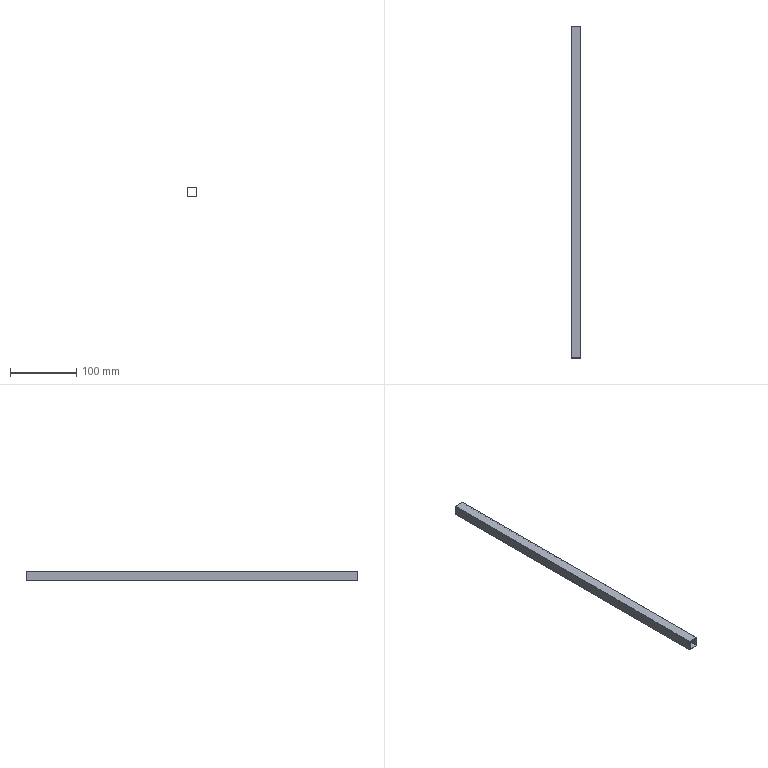Component | SolidWorks | Column-2 | 1 solid | 10 faces | box 15 x 500 x 15 mm | volume 28000 mm3 | plane 10
build123d program:
from build123d import *

# Parameters (mm, degrees)
SKETCH1_W           = 15
SKETCH1_H           = 15
SKETCH1_W_2         = 13
SKETCH1_H_2         = 13
BOSS_EXTRUDE1_DEPTH = 500


with BuildPart() as part:
    # Sketch1 → Boss-Extrude1 (new body)
    with BuildSketch(Plane(origin=(0, 0, 0), x_dir=(1, 0, 0), z_dir=(0, 1, 0))):
        Rectangle(SKETCH1_W, SKETCH1_H)
        Rectangle(SKETCH1_W_2, SKETCH1_H_2, mode=Mode.SUBTRACT)
    extrude(amount=BOSS_EXTRUDE1_DEPTH)


solid = part.part

# Placed as in the assembly
solid = solid.moved(Location((75.741, -541.715, 1459.224), (0, 0, 0)))
STEP:
#1=COLOUR_RGB('',0.7922,0.8196,0.9333);
#2=FILL_AREA_STYLE_COLOUR('',#1);
#3=FILL_AREA_STYLE('',(#2));
#4=SURFACE_STYLE_FILL_AREA(#3);
#5=SURFACE_SIDE_STYLE('',(#4));
#6=SURFACE_STYLE_USAGE(.BOTH.,#5);
#7=PRESENTATION_STYLE_ASSIGNMENT((#6));
#8=CARTESIAN_POINT('',(2.687,-1.642,57.155));
#9=VERTEX_POINT('',#8);
#10=CARTESIAN_POINT('',(2.687,-1.642,57.745));
#11=VERTEX_POINT('',#10);
#12=CARTESIAN_POINT('',(2.687,-1.642,57.155));
#13=DIRECTION('',(0.,0.,1.));
#14=VECTOR('',#13,39.37);
#15=LINE('',#12,#14);
#16=EDGE_CURVE('',#9,#11,#15,.T.);
#17=ORIENTED_EDGE('',*,*,#16,.T.);
#18=CARTESIAN_POINT('',(3.277,-1.642,57.745));
#19=VERTEX_POINT('',#18);
#20=CARTESIAN_POINT('',(3.277,-1.642,57.745));
#21=DIRECTION('',(1.,0.,0.));
#22=VECTOR('',#21,39.37);
#23=LINE('',#20,#22);
#24=EDGE_CURVE('',#11,#19,#23,.T.);
#25=ORIENTED_EDGE('',*,*,#24,.T.);
#26=CARTESIAN_POINT('',(3.277,-1.642,57.155));
#27=VERTEX_POINT('',#26);
#28=CARTESIAN_POINT('',(3.277,-1.642,57.155));
#29=DIRECTION('',(0.,0.,-1.));
#30=VECTOR('',#29,39.37);
#31=LINE('',#28,#30);
#32=EDGE_CURVE('',#19,#27,#31,.T.);
#33=ORIENTED_EDGE('',*,*,#32,.T.);
#34=CARTESIAN_POINT('',(3.277,-1.642,57.155));
#35=DIRECTION('',(-1.,0.,0.));
#36=VECTOR('',#35,39.37);
#37=LINE('',#34,#36);
#38=EDGE_CURVE('',#27,#9,#37,.T.);
#39=ORIENTED_EDGE('',*,*,#38,.T.);
#40=EDGE_LOOP('',(#17,#25,#33,#39));
#41=FACE_OUTER_BOUND('',#40,.T.);
#42=CARTESIAN_POINT('',(3.238,-1.642,57.706));
#43=VERTEX_POINT('',#42);
#44=CARTESIAN_POINT('',(3.238,-1.642,57.194));
#45=VERTEX_POINT('',#44);
#46=CARTESIAN_POINT('',(3.238,-1.642,57.194));
#47=DIRECTION('',(0.,0.,-1.));
#48=VECTOR('',#47,39.37);
#49=LINE('',#46,#48);
#50=EDGE_CURVE('',#43,#45,#49,.T.);
#51=ORIENTED_EDGE('',*,*,#50,.F.);
#52=CARTESIAN_POINT('',(2.726,-1.642,57.706));
#53=VERTEX_POINT('',#52);
#54=CARTESIAN_POINT('',(2.726,-1.642,57.706));
#55=DIRECTION('',(1.,0.,0.));
#56=VECTOR('',#55,39.37);
#57=LINE('',#54,#56);
#58=EDGE_CURVE('',#53,#43,#57,.T.);
#59=ORIENTED_EDGE('',*,*,#58,.F.);
#60=CARTESIAN_POINT('',(2.726,-1.642,57.194));
#61=VERTEX_POINT('',#60);
#62=CARTESIAN_POINT('',(2.726,-1.642,57.194));
#63=DIRECTION('',(0.,0.,1.));
#64=VECTOR('',#63,39.37);
#65=LINE('',#62,#64);
#66=EDGE_CURVE('',#61,#53,#65,.T.);
#67=ORIENTED_EDGE('',*,*,#66,.F.);
#68=CARTESIAN_POINT('',(2.726,-1.642,57.194));
#69=DIRECTION('',(-1.,0.,-0.));
#70=VECTOR('',#69,39.37);
#71=LINE('',#68,#70);
#72=EDGE_CURVE('',#45,#61,#71,.T.);
#73=ORIENTED_EDGE('',*,*,#72,.F.);
#74=EDGE_LOOP('',(#51,#59,#67,#73));
#75=FACE_BOUND('',#74,.T.);
#76=CARTESIAN_POINT('',(2.982,-1.642,57.45));
#77=DIRECTION('',(0.,-1.,0.));
#78=DIRECTION('',(0.,0.,1.));
#79=AXIS2_PLACEMENT_3D('',#76,#77,#78);
#80=PLANE('',#79);
#81=ADVANCED_FACE('',(#41,#75),#80,.F.);
#82=CARTESIAN_POINT('',(2.687,-21.327,57.155));
#83=VERTEX_POINT('',#82);
#84=CARTESIAN_POINT('',(2.687,-21.327,57.745));
#85=VERTEX_POINT('',#84);
#86=CARTESIAN_POINT('',(2.687,-21.327,57.155));
#87=DIRECTION('',(0.,0.,1.));
#88=VECTOR('',#87,39.37);
#89=LINE('',#86,#88);
#90=EDGE_CURVE('',#83,#85,#89,.T.);
#91=ORIENTED_EDGE('',*,*,#90,.F.);
#92=CARTESIAN_POINT('',(3.277,-21.327,57.155));
#93=VERTEX_POINT('',#92);
#94=CARTESIAN_POINT('',(3.277,-21.327,57.155));
#95=DIRECTION('',(-1.,0.,0.));
#96=VECTOR('',#95,39.37);
#97=LINE('',#94,#96);
#98=EDGE_CURVE('',#93,#83,#97,.T.);
#99=ORIENTED_EDGE('',*,*,#98,.F.);
#100=CARTESIAN_POINT('',(3.277,-21.327,57.745));
#101=VERTEX_POINT('',#100);
#102=CARTESIAN_POINT('',(3.277,-21.327,57.155));
#103=DIRECTION('',(0.,0.,-1.));
#104=VECTOR('',#103,39.37);
#105=LINE('',#102,#104);
#106=EDGE_CURVE('',#101,#93,#105,.T.);
#107=ORIENTED_EDGE('',*,*,#106,.F.);
#108=CARTESIAN_POINT('',(3.277,-21.327,57.745));
#109=DIRECTION('',(1.,0.,0.));
#110=VECTOR('',#109,39.37);
#111=LINE('',#108,#110);
#112=EDGE_CURVE('',#85,#101,#111,.T.);
#113=ORIENTED_EDGE('',*,*,#112,.F.);
#114=EDGE_LOOP('',(#91,#99,#107,#113));
#115=FACE_OUTER_BOUND('',#114,.T.);
#116=CARTESIAN_POINT('',(2.726,-21.327,57.706));
#117=VERTEX_POINT('',#116);
#118=CARTESIAN_POINT('',(3.238,-21.327,57.706));
#119=VERTEX_POINT('',#118);
#120=CARTESIAN_POINT('',(2.726,-21.327,57.706));
#121=DIRECTION('',(1.,0.,0.));
#122=VECTOR('',#121,39.37);
#123=LINE('',#120,#122);
#124=EDGE_CURVE('',#117,#119,#123,.T.);
#125=ORIENTED_EDGE('',*,*,#124,.T.);
#126=CARTESIAN_POINT('',(3.238,-21.327,57.194));
#127=VERTEX_POINT('',#126);
#128=CARTESIAN_POINT('',(3.238,-21.327,57.194));
#129=DIRECTION('',(0.,0.,-1.));
#130=VECTOR('',#129,39.37);
#131=LINE('',#128,#130);
#132=EDGE_CURVE('',#119,#127,#131,.T.);
#133=ORIENTED_EDGE('',*,*,#132,.T.);
#134=CARTESIAN_POINT('',(2.726,-21.327,57.194));
#135=VERTEX_POINT('',#134);
#136=CARTESIAN_POINT('',(2.726,-21.327,57.194));
#137=DIRECTION('',(-1.,0.,-0.));
#138=VECTOR('',#137,39.37);
#139=LINE('',#136,#138);
#140=EDGE_CURVE('',#127,#135,#139,.T.);
#141=ORIENTED_EDGE('',*,*,#140,.T.);
#142=CARTESIAN_POINT('',(2.726,-21.327,57.194));
#143=DIRECTION('',(0.,0.,1.));
#144=VECTOR('',#143,39.37);
#145=LINE('',#142,#144);
#146=EDGE_CURVE('',#135,#117,#145,.T.);
#147=ORIENTED_EDGE('',*,*,#146,.T.);
#148=EDGE_LOOP('',(#125,#133,#141,#147));
#149=FACE_BOUND('',#148,.T.);
#150=CARTESIAN_POINT('',(2.982,-21.327,57.45));
#151=DIRECTION('',(0.,-1.,0.));
#152=DIRECTION('',(0.,0.,1.));
#153=AXIS2_PLACEMENT_3D('',#150,#151,#152);
#154=PLANE('',#153);
#155=ADVANCED_FACE('',(#115,#149),#154,.T.);
#156=ORIENTED_EDGE('',*,*,#90,.T.);
#157=CARTESIAN_POINT('',(2.687,-1.642,57.745));
#158=DIRECTION('',(0.,-1.,0.));
#159=VECTOR('',#158,39.37);
#160=LINE('',#157,#159);
#161=EDGE_CURVE('',#11,#85,#160,.T.);
#162=ORIENTED_EDGE('',*,*,#161,.F.);
#163=ORIENTED_EDGE('',*,*,#16,.F.);
#164=CARTESIAN_POINT('',(2.687,-1.642,57.155));
#165=DIRECTION('',(0.,-1.,0.));
#166=VECTOR('',#165,39.37);
#167=LINE('',#164,#166);
#168=EDGE_CURVE('',#9,#83,#167,.T.);
#169=ORIENTED_EDGE('',*,*,#168,.T.);
#170=EDGE_LOOP('',(#156,#162,#163,#169));
#171=FACE_OUTER_BOUND('',#170,.T.);
#172=CARTESIAN_POINT('',(2.687,-1.642,57.155));
#173=DIRECTION('',(1.,0.,0.));
#174=DIRECTION('',(0.,0.,-1.));
#175=AXIS2_PLACEMENT_3D('',#172,#173,#174);
#176=PLANE('',#175);
#177=ADVANCED_FACE('',(#171),#176,.F.);
#178=ORIENTED_EDGE('',*,*,#112,.T.);
#179=CARTESIAN_POINT('',(3.277,-1.642,57.745));
#180=DIRECTION('',(0.,-1.,0.));
#181=VECTOR('',#180,39.37);
#182=LINE('',#179,#181);
#183=EDGE_CURVE('',#19,#101,#182,.T.);
#184=ORIENTED_EDGE('',*,*,#183,.F.);
#185=ORIENTED_EDGE('',*,*,#24,.F.);
#186=ORIENTED_EDGE('',*,*,#161,.T.);
#187=EDGE_LOOP('',(#178,#184,#185,#186));
#188=FACE_OUTER_BOUND('',#187,.T.);
#189=CARTESIAN_POINT('',(3.277,-1.642,57.745));
#190=DIRECTION('',(0.,0.,-1.));
#191=DIRECTION('',(-1.,0.,0.));
#192=AXIS2_PLACEMENT_3D('',#189,#190,#191);
#193=PLANE('',#192);
#194=ADVANCED_FACE('',(#188),#193,.F.);
#195=ORIENTED_EDGE('',*,*,#106,.T.);
#196=CARTESIAN_POINT('',(3.277,-1.642,57.155));
#197=DIRECTION('',(0.,-1.,0.));
#198=VECTOR('',#197,39.37);
#199=LINE('',#196,#198);
#200=EDGE_CURVE('',#27,#93,#199,.T.);
#201=ORIENTED_EDGE('',*,*,#200,.F.);
#202=ORIENTED_EDGE('',*,*,#32,.F.);
#203=ORIENTED_EDGE('',*,*,#183,.T.);
#204=EDGE_LOOP('',(#195,#201,#202,#203));
#205=FACE_OUTER_BOUND('',#204,.T.);
#206=CARTESIAN_POINT('',(3.277,-1.642,57.155));
#207=DIRECTION('',(-1.,0.,0.));
#208=DIRECTION('',(0.,0.,1.));
#209=AXIS2_PLACEMENT_3D('',#206,#207,#208);
#210=PLANE('',#209);
#211=ADVANCED_FACE('',(#205),#210,.F.);
#212=ORIENTED_EDGE('',*,*,#98,.T.);
#213=ORIENTED_EDGE('',*,*,#168,.F.);
#214=ORIENTED_EDGE('',*,*,#38,.F.);
#215=ORIENTED_EDGE('',*,*,#200,.T.);
#216=EDGE_LOOP('',(#212,#213,#214,#215));
#217=FACE_OUTER_BOUND('',#216,.T.);
#218=CARTESIAN_POINT('',(3.277,-1.642,57.155));
#219=DIRECTION('',(0.,0.,1.));
#220=DIRECTION('',(1.,0.,0.));
#221=AXIS2_PLACEMENT_3D('',#218,#219,#220);
#222=PLANE('',#221);
#223=ADVANCED_FACE('',(#217),#222,.F.);
#224=ORIENTED_EDGE('',*,*,#132,.F.);
#225=CARTESIAN_POINT('',(3.238,-1.642,57.706));
#226=DIRECTION('',(0.,-1.,0.));
#227=VECTOR('',#226,39.37);
#228=LINE('',#225,#227);
#229=EDGE_CURVE('',#43,#119,#228,.T.);
#230=ORIENTED_EDGE('',*,*,#229,.F.);
#231=ORIENTED_EDGE('',*,*,#50,.T.);
#232=CARTESIAN_POINT('',(3.238,-1.642,57.194));
#233=DIRECTION('',(0.,-1.,0.));
#234=VECTOR('',#233,39.37);
#235=LINE('',#232,#234);
#236=EDGE_CURVE('',#45,#127,#235,.T.);
#237=ORIENTED_EDGE('',*,*,#236,.T.);
#238=EDGE_LOOP('',(#224,#230,#231,#237));
#239=FACE_OUTER_BOUND('',#238,.T.);
#240=CARTESIAN_POINT('',(3.238,-1.642,57.194));
#241=DIRECTION('',(-1.,0.,0.));
#242=DIRECTION('',(0.,0.,1.));
#243=AXIS2_PLACEMENT_3D('',#240,#241,#242);
#244=PLANE('',#243);
#245=ADVANCED_FACE('',(#239),#244,.T.);
#246=ORIENTED_EDGE('',*,*,#140,.F.);
#247=ORIENTED_EDGE('',*,*,#236,.F.);
#248=ORIENTED_EDGE('',*,*,#72,.T.);
#249=CARTESIAN_POINT('',(2.726,-1.642,57.194));
#250=DIRECTION('',(0.,-1.,0.));
#251=VECTOR('',#250,39.37);
#252=LINE('',#249,#251);
#253=EDGE_CURVE('',#61,#135,#252,.T.);
#254=ORIENTED_EDGE('',*,*,#253,.T.);
#255=EDGE_LOOP('',(#246,#247,#248,#254));
#256=FACE_OUTER_BOUND('',#255,.T.);
#257=CARTESIAN_POINT('',(2.726,-1.642,57.194));
#258=DIRECTION('',(-0.,0.,1.));
#259=DIRECTION('',(1.,0.,0.));
#260=AXIS2_PLACEMENT_3D('',#257,#258,#259);
#261=PLANE('',#260);
#262=ADVANCED_FACE('',(#256),#261,.T.);
#263=ORIENTED_EDGE('',*,*,#146,.F.);
#264=ORIENTED_EDGE('',*,*,#253,.F.);
#265=ORIENTED_EDGE('',*,*,#66,.T.);
#266=CARTESIAN_POINT('',(2.726,-1.642,57.706));
#267=DIRECTION('',(0.,-1.,0.));
#268=VECTOR('',#267,39.37);
#269=LINE('',#266,#268);
#270=EDGE_CURVE('',#53,#117,#269,.T.);
#271=ORIENTED_EDGE('',*,*,#270,.T.);
#272=EDGE_LOOP('',(#263,#264,#265,#271));
#273=FACE_OUTER_BOUND('',#272,.T.);
#274=CARTESIAN_POINT('',(2.726,-1.642,57.194));
#275=DIRECTION('',(1.,0.,-0.));
#276=DIRECTION('',(-0.,0.,-1.));
#277=AXIS2_PLACEMENT_3D('',#274,#275,#276);
#278=PLANE('',#277);
#279=ADVANCED_FACE('',(#273),#278,.T.);
#280=ORIENTED_EDGE('',*,*,#124,.F.);
#281=ORIENTED_EDGE('',*,*,#270,.F.);
#282=ORIENTED_EDGE('',*,*,#58,.T.);
#283=ORIENTED_EDGE('',*,*,#229,.T.);
#284=EDGE_LOOP('',(#280,#281,#282,#283));
#285=FACE_OUTER_BOUND('',#284,.T.);
#286=CARTESIAN_POINT('',(2.726,-1.642,57.706));
#287=DIRECTION('',(0.,0.,-1.));
#288=DIRECTION('',(-1.,0.,0.));
#289=AXIS2_PLACEMENT_3D('',#286,#287,#288);
#290=PLANE('',#289);
#291=ADVANCED_FACE('',(#285),#290,.T.);
#292=CLOSED_SHELL('',(#81,#155,#177,#194,#211,#223,#245,#262,#279,#291));
#293=MANIFOLD_SOLID_BREP('',#292);
#294=STYLED_ITEM('',(#7),#293);
#295=(LENGTH_UNIT()NAMED_UNIT(*)SI_UNIT($,.METRE.));
#296=LENGTH_MEASURE_WITH_UNIT(LENGTH_MEASURE(0.0254),#295);
#297=DIMENSIONAL_EXPONENTS(1.,0.,0.,0.,0.,0.,0.);
#298=(CONVERSION_BASED_UNIT('',#296)LENGTH_UNIT()NAMED_UNIT(#297));
#299=UNCERTAINTY_MEASURE_WITH_UNIT(LENGTH_MEASURE(0.00001),#298,'','');
#300=(NAMED_UNIT(*)PLANE_ANGLE_UNIT()SI_UNIT($,.RADIAN.));
#301=(NAMED_UNIT(*)SI_UNIT($,.STERADIAN.)SOLID_ANGLE_UNIT());
#302=(GEOMETRIC_REPRESENTATION_CONTEXT(3)GLOBAL_UNCERTAINTY_ASSIGNED_CONTEXT((#299))GLOBAL_UNIT_ASSIGNED_CONTEXT((#298,#300,#301))REPRESENTATION_CONTEXT('',''));
#303=MECHANICAL_DESIGN_GEOMETRIC_PRESENTATION_REPRESENTATION('',(#294),#302);
#304=CARTESIAN_POINT('',(0.,0.,0.));
#305=DIRECTION('',(0.,0.,1.));
#306=DIRECTION('',(1.,0.,0.));
#307=AXIS2_PLACEMENT_3D('',#304,#305,#306);
#308=(LENGTH_UNIT()NAMED_UNIT(*)SI_UNIT($,.METRE.));
#309=LENGTH_MEASURE_WITH_UNIT(LENGTH_MEASURE(0.0254),#308);
#310=DIMENSIONAL_EXPONENTS(1.,0.,0.,0.,0.,0.,0.);
#311=(CONVERSION_BASED_UNIT('',#309)LENGTH_UNIT()NAMED_UNIT(#310));
#312=UNCERTAINTY_MEASURE_WITH_UNIT(LENGTH_MEASURE(0.00001),#311,'','');
#313=(NAMED_UNIT(*)PLANE_ANGLE_UNIT()SI_UNIT($,.RADIAN.));
#314=(NAMED_UNIT(*)SI_UNIT($,.STERADIAN.)SOLID_ANGLE_UNIT());
#315=(GEOMETRIC_REPRESENTATION_CONTEXT(3)GLOBAL_UNCERTAINTY_ASSIGNED_CONTEXT((#312))GLOBAL_UNIT_ASSIGNED_CONTEXT((#311,#313,#314))REPRESENTATION_CONTEXT('',''));
#316=ADVANCED_BREP_SHAPE_REPRESENTATION('',(#293,#307),#315);
#317=PRESENTATION_LAYER_ASSIGNMENT('','',(#294));